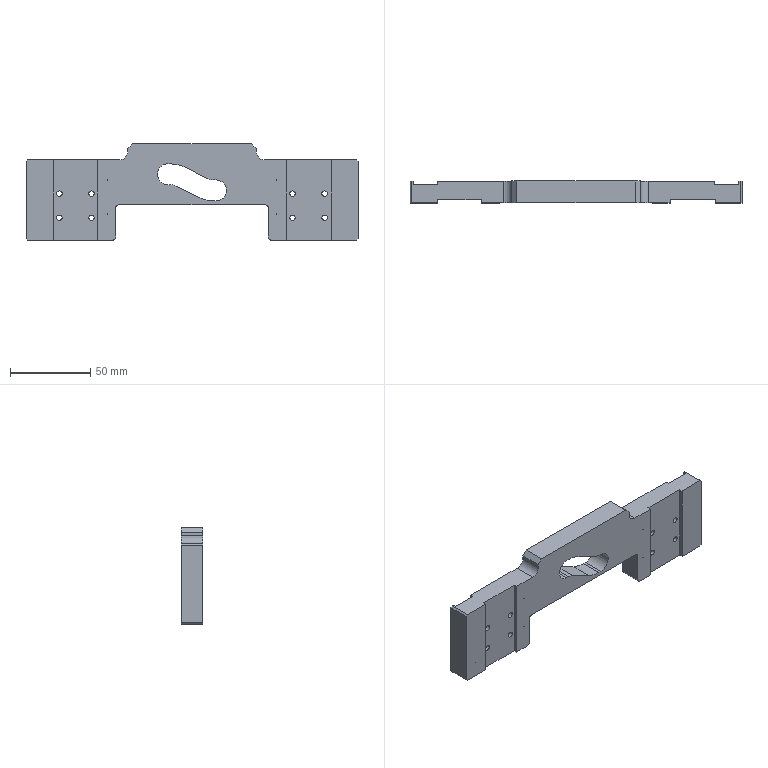Component | SolidWorks | 12-DividingMechanism-1111-1_14-Z1-1111-1 | 1 solid | 127 faces | box 206.5 x 13.6 x 60 mm | volume 104322 mm3 | cylinder 61 | plane 50 | cone 16 | commonest cylinder face diameters 6.5 x16 3.4 x16 4.2 x8 3.3 x8 4 x4 13 x3 41 x2 15 x2
build123d program:
from build123d import *

# Parameters (mm, degrees)
SKETCH5_W                                       = 60
SKETCH5_H                                       = 206.5
BOSS_EXTRUDE1_DEPTH                             = 13.6
SKETCH11_W                                      = 60
SKETCH11_H                                      = 27
CUT_EXTRUDE4_DEPTH                              = 2
SKETCH12_W                                      = 10
SKETCH12_H                                      = 63.25
CUT_EXTRUDE5_DEPTH                              = 109.377
CUT_EXTRUDE6_DEPTH                              = 109.377
SKETCH14_W                                      = 50
SKETCH14_H                                      = 15
CUT_EXTRUDE7_DEPTH                              = 2
SKETCH15_W                                      = 44
SKETCH15_H                                      = 95
CUT_EXTRUDE8_DEPTH                              = 109.377
FILLET1_R                                       = 2
CHAMFER1_SIZE                                   = 1
FILLET2_R                                       = 5
CHAMFER2_SIZE                                   = 3
M3_HEX_SOCKET_HEAD_CAP_SCREW_CBORE1_D           = 3.4
M3_HEX_SOCKET_HEAD_CAP_SCREW_CBORE1_CBORE_D     = 6.5
M3_HEX_SOCKET_HEAD_CAP_SCREW_CBORE1_CBORE_DEPTH = 3.4
M4_TAPPED_HOLE1_D                               = 3.3
M4_TAPPED_HOLE1_DEPTH                           = 10.1
M4_TAPPED_HOLE1_TIP                             = 0.9914
M5_TAPPED_HOLE1_D                               = 4.2
M5_TAPPED_HOLE1_DEPTH                           = 12.4
M5_TAPPED_HOLE1_TIP                             = 1.262
MOVE_FACE1_BY                                   = 0.5
MOVE_FACE2_BY                                   = 0.5


with BuildPart() as part:
    # Sketch5 → Boss-Extrude1 (new body)
    with BuildSketch(Plane(origin=(0, 0, 0), x_dir=(1, 0, 0), z_dir=(0, 1, 0))):
        Rectangle(SKETCH5_W, SKETCH5_H)
    extrude(amount=BOSS_EXTRUDE1_DEPTH)

    # Sketch11 → Cut-Extrude4 (cut)
    with BuildSketch(Plane.XZ):
        with Locations((0, 72.5)):
            Rectangle(SKETCH11_W, SKETCH11_H)
        with Locations((0, -72.5)):
            Rectangle(SKETCH11_W, SKETCH11_H)
    extrude(amount=-CUT_EXTRUDE4_DEPTH, mode=Mode.SUBTRACT)

    # Sketch12 → Cut-Extrude5 (cut, through all)
    with BuildSketch(Plane(origin=(0, 13.6, 0), x_dir=(1, 0, 0), z_dir=(0, 1, 0))):
        with Locations((25, 71.625)):
            Rectangle(SKETCH12_W, SKETCH12_H)
        with Locations((25, -71.625)):
            Rectangle(SKETCH12_W, SKETCH12_H)
    extrude(amount=-CUT_EXTRUDE5_DEPTH, mode=Mode.SUBTRACT)

    # Sketch13 → Cut-Extrude6 (cut, through all)
    with BuildSketch(Plane(origin=(0, 13.6, 0), x_dir=(1, 0, 0), z_dir=(0, 1, 0))):
        with BuildLine():
            Line((-5.5, 13.305), (-5.5, 15))
            ThreePointArc((-5.5, 15), (1, 21.5), (7.5, 15))
            Line((7.5, 15), (7.5, 13.305))
            ThreePointArc((7.5, 13.305), (7.701, 11.582), (8.292, 9.951))
            Line((8.292, 9.951), (15.336, -4.137))
            ThreePointArc((15.336, -4.137), (16.952, -8.595), (17.5, -13.305))
            Line((17.5, -13.305), (17.5, -15))
            ThreePointArc((17.5, -15), (11, -21.5), (4.5, -15))
            Line((4.5, -15), (4.5, -13.305))
            ThreePointArc((4.5, -13.305), (4.299, -11.582), (3.708, -9.951))
            Line((3.708, -9.951), (-3.336, 4.137))
            ThreePointArc((-3.336, 4.137), (-4.952, 8.595), (-5.5, 13.305))
        make_face()
    extrude(amount=-CUT_EXTRUDE6_DEPTH, mode=Mode.SUBTRACT)

    # Sketch14 → Cut-Extrude7 (cut)
    with BuildSketch(Plane(origin=(0, 13.6, 0), x_dir=(1, 0, 0), z_dir=(0, 1, 0))):
        with Locations((-5, -93.75)):
            Rectangle(SKETCH14_W, SKETCH14_H)
        with Locations((-5, 93.75)):
            Rectangle(SKETCH14_W, SKETCH14_H)
    extrude(amount=-CUT_EXTRUDE7_DEPTH, mode=Mode.SUBTRACT)

    # Sketch15 → Cut-Extrude8 (cut, through all)
    with BuildSketch(Plane(origin=(0, 13.6, 0), x_dir=(1, 0, 0), z_dir=(0, 1, 0))):
        with Locations((-30, 0)):
            Rectangle(SKETCH15_W, SKETCH15_H)
    extrude(amount=-CUT_EXTRUDE8_DEPTH, mode=Mode.SUBTRACT)

    # Fillet1
    fillet1_edges = [part.edges().sort_by_distance(p)[0] for p in [
        (-30, 6.8, 47.5),
        (-8, 6.8, 47.5),
        (-30, 6.8, -47.5),
        (-8, 6.8, -47.5),
    ]]
    fillet(fillet1_edges, radius=FILLET1_R)

    # Chamfer1
    chamfer1_edges = [part.edges().sort_by_distance(p)[0] for p in [
        (20, 6.8, 103.25),
        (-30, 6.8, -103.25),
        (20, 6.8, -103.25),
        (-30, 6.8, 103.25),
    ]]
    chamfer(chamfer1_edges, length=CHAMFER1_SIZE)

    # Fillet2
    fillet2_edges = [part.edges().sort_by_distance(p)[0] for p in [
        (20, 6.8, 40),
        (20, 6.8, -40),
    ]]
    fillet(fillet2_edges, radius=FILLET2_R)

    # Chamfer2
    chamfer2_edges = [part.edges().sort_by_distance(p)[0] for p in [
        (30, 6.8, 40),
        (30, 6.8, -40),
    ]]
    chamfer(chamfer2_edges, length=CHAMFER2_SIZE)

    # M3 Hex Socket Head Cap Screw CBORE1 (through all)
    with Locations(Plane(origin=(0, 13.6, 0), x_dir=(1, 0, 0), z_dir=(0, 1, 0))):
        with Locations((-16, -62.5), (-16, -82.5), (-1, -82.5), (-1, -62.5)):
            m3_hex_socket_head_cap_screw_cbore1 = CounterBoreHole(M3_HEX_SOCKET_HEAD_CAP_SCREW_CBORE1_D / 2, M3_HEX_SOCKET_HEAD_CAP_SCREW_CBORE1_CBORE_D / 2, M3_HEX_SOCKET_HEAD_CAP_SCREW_CBORE1_CBORE_DEPTH)

    # Mirror1: M3 Hex Socket Head Cap Screw CBORE1 across plane
    add(m3_hex_socket_head_cap_screw_cbore1.mirror(Plane.XY), mode=Mode.SUBTRACT)

    # M4 Tapped Hole1
    with Locations(Plane(origin=(0, 11.6, 0), x_dir=(1, 0, 0), z_dir=(0, 1, 0))):
        with Locations((10, 93.75), (-20, 93.75), (10, -93.75), (-20, -94.787)):
            Hole(M4_TAPPED_HOLE1_D / 2, depth=M4_TAPPED_HOLE1_DEPTH)
            with Locations((0, 0, -(M4_TAPPED_HOLE1_DEPTH + M4_TAPPED_HOLE1_TIP / 2))):  # 118° drill point
                Cone(0, M4_TAPPED_HOLE1_D / 2, M4_TAPPED_HOLE1_TIP, mode=Mode.SUBTRACT)

    # M5 Tapped Hole1
    with Locations(Plane(origin=(0, 13.6, 0), x_dir=(1, 0, 0), z_dir=(0, 1, 0))):
        with Locations((-13.6, 52.5), (7.4, 52.5), (7.4, -52.5), (-13.6, -52.5)):
            Hole(M5_TAPPED_HOLE1_D / 2, depth=M5_TAPPED_HOLE1_DEPTH)
            with Locations((0, 0, -(M5_TAPPED_HOLE1_DEPTH + M5_TAPPED_HOLE1_TIP / 2))):  # 118° drill point
                Cone(0, M5_TAPPED_HOLE1_D / 2, M5_TAPPED_HOLE1_TIP, mode=Mode.SUBTRACT)

    # Move Face1: a face moved inward by 0.5
    extrude(part.faces().sort_by_distance((-5, 1, -86))[0], amount=MOVE_FACE1_BY, dir=(0, 0, -1), mode=Mode.SUBTRACT)

    # Move Face2: a face moved inward by 0.5
    extrude(part.faces().sort_by_distance((-5, 1, -59))[0], amount=MOVE_FACE2_BY, dir=(0, 0, 1), mode=Mode.SUBTRACT)


solid = part.part

# Placed as in the assembly
solid = solid.moved(Location((3.428, 560.224, 1534.056), (0, -90, 0)))